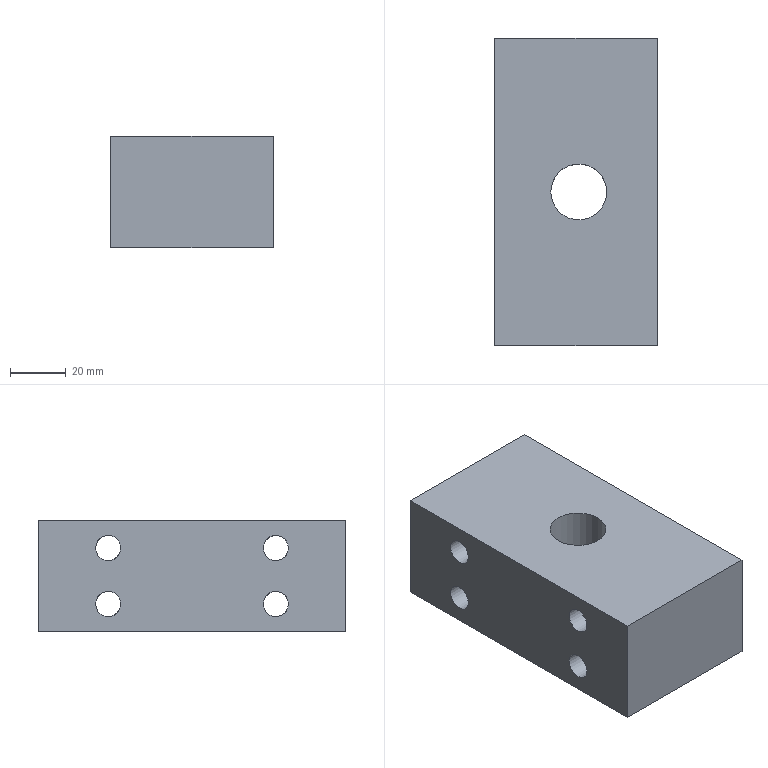Component | NX | CH3404_2-3 | 1 solid | 11 faces | box 58 x 110 x 40 mm | volume 227874 mm3 | plane 6 | cylinder 5 | commonest cylinder face diameters 9 x4 20 x1
STEP:
#1=CARTESIAN_POINT('',(0.,0.,0.));
#2=DIRECTION('',(0.,0.,1.));
#3=DIRECTION('',(1.,0.,0.));
#4=AXIS2_PLACEMENT_3D('',#1,#2,#3);
#5=CARTESIAN_POINT('',(0.,30.,5.5));
#6=VERTEX_POINT('',#5);
#7=CARTESIAN_POINT('',(0.,30.,10.));
#8=DIRECTION('',(1.,0.,0.));
#9=DIRECTION('',(0.,0.,-1.));
#10=AXIS2_PLACEMENT_3D('',#7,#8,#9);
#11=CIRCLE('',#10,4.5);
#12=CARTESIAN_POINT('',(-0.,55.,20.));
#13=DIRECTION('',(1.,0.,0.));
#14=DIRECTION('',(0.,0.,-1.));
#15=AXIS2_PLACEMENT_3D('',#12,#13,#14);
#16=PLANE('',#15);
#17=CARTESIAN_POINT('',(10.,-25.));
#18=DIRECTION('',(1.,0.));
#19=AXIS2_PLACEMENT_2D('',#17,#18);
#20=CIRCLE('',#19,4.5);
#21=(GEOMETRIC_REPRESENTATION_CONTEXT(2)PARAMETRIC_REPRESENTATION_CONTEXT()REPRESENTATION_CONTEXT('',''));
#22=DEFINITIONAL_REPRESENTATION('',(#20),#21);
#23=PCURVE('',#16,#22);
#24=CARTESIAN_POINT('',(0.,30.,10.));
#25=DIRECTION('',(1.,0.,0.));
#26=DIRECTION('',(0.,0.,-1.));
#27=AXIS2_PLACEMENT_3D('',#24,#25,#26);
#28=CYLINDRICAL_SURFACE('',#27,4.5);
#29=CARTESIAN_POINT('',(0.,0.));
#30=DIRECTION('',(1.,0.));
#31=VECTOR('',#30,1.);
#32=LINE('',#29,#31);
#33=(GEOMETRIC_REPRESENTATION_CONTEXT(2)PARAMETRIC_REPRESENTATION_CONTEXT()REPRESENTATION_CONTEXT('',''));
#34=DEFINITIONAL_REPRESENTATION('',(#32),#33);
#35=PCURVE('',#28,#34);
#36=SURFACE_CURVE('',#11,(#23,#35),.PCURVE_S1.);
#37=EDGE_CURVE('',#6,#6,#36,.T.);
#38=ORIENTED_EDGE('',*,*,#37,.T.);
#39=EDGE_LOOP('',(#38));
#40=FACE_BOUND('',#39,.T.);
#41=CARTESIAN_POINT('',(0.,30.,-14.5));
#42=VERTEX_POINT('',#41);
#43=CARTESIAN_POINT('',(0.,30.,-10.));
#44=DIRECTION('',(1.,0.,0.));
#45=DIRECTION('',(0.,0.,-1.));
#46=AXIS2_PLACEMENT_3D('',#43,#44,#45);
#47=CIRCLE('',#46,4.5);
#48=CARTESIAN_POINT('',(30.,-25.));
#49=DIRECTION('',(1.,0.));
#50=AXIS2_PLACEMENT_2D('',#48,#49);
#51=CIRCLE('',#50,4.5);
#52=(GEOMETRIC_REPRESENTATION_CONTEXT(2)PARAMETRIC_REPRESENTATION_CONTEXT()REPRESENTATION_CONTEXT('',''));
#53=DEFINITIONAL_REPRESENTATION('',(#51),#52);
#54=PCURVE('',#16,#53);
#55=CARTESIAN_POINT('',(0.,30.,-10.));
#56=DIRECTION('',(1.,0.,0.));
#57=DIRECTION('',(0.,0.,-1.));
#58=AXIS2_PLACEMENT_3D('',#55,#56,#57);
#59=CYLINDRICAL_SURFACE('',#58,4.5);
#60=CARTESIAN_POINT('',(0.,0.));
#61=DIRECTION('',(1.,0.));
#62=VECTOR('',#61,1.);
#63=LINE('',#60,#62);
#64=(GEOMETRIC_REPRESENTATION_CONTEXT(2)PARAMETRIC_REPRESENTATION_CONTEXT()REPRESENTATION_CONTEXT('',''));
#65=DEFINITIONAL_REPRESENTATION('',(#63),#64);
#66=PCURVE('',#59,#65);
#67=SURFACE_CURVE('',#47,(#54,#66),.PCURVE_S1.);
#68=EDGE_CURVE('',#42,#42,#67,.T.);
#69=ORIENTED_EDGE('',*,*,#68,.T.);
#70=EDGE_LOOP('',(#69));
#71=FACE_BOUND('',#70,.T.);
#72=CARTESIAN_POINT('',(0.,-30.,5.5));
#73=VERTEX_POINT('',#72);
#74=CARTESIAN_POINT('',(0.,-30.,10.));
#75=DIRECTION('',(1.,0.,0.));
#76=DIRECTION('',(0.,0.,-1.));
#77=AXIS2_PLACEMENT_3D('',#74,#75,#76);
#78=CIRCLE('',#77,4.5);
#79=CARTESIAN_POINT('',(10.,-85.));
#80=DIRECTION('',(1.,0.));
#81=AXIS2_PLACEMENT_2D('',#79,#80);
#82=CIRCLE('',#81,4.5);
#83=(GEOMETRIC_REPRESENTATION_CONTEXT(2)PARAMETRIC_REPRESENTATION_CONTEXT()REPRESENTATION_CONTEXT('',''));
#84=DEFINITIONAL_REPRESENTATION('',(#82),#83);
#85=PCURVE('',#16,#84);
#86=CARTESIAN_POINT('',(0.,-30.,10.));
#87=DIRECTION('',(1.,0.,0.));
#88=DIRECTION('',(0.,0.,-1.));
#89=AXIS2_PLACEMENT_3D('',#86,#87,#88);
#90=CYLINDRICAL_SURFACE('',#89,4.5);
#91=CARTESIAN_POINT('',(0.,0.));
#92=DIRECTION('',(1.,0.));
#93=VECTOR('',#92,1.);
#94=LINE('',#91,#93);
#95=(GEOMETRIC_REPRESENTATION_CONTEXT(2)PARAMETRIC_REPRESENTATION_CONTEXT()REPRESENTATION_CONTEXT('',''));
#96=DEFINITIONAL_REPRESENTATION('',(#94),#95);
#97=PCURVE('',#90,#96);
#98=SURFACE_CURVE('',#78,(#85,#97),.PCURVE_S1.);
#99=EDGE_CURVE('',#73,#73,#98,.T.);
#100=ORIENTED_EDGE('',*,*,#99,.T.);
#101=EDGE_LOOP('',(#100));
#102=FACE_BOUND('',#101,.T.);
#103=CARTESIAN_POINT('',(0.,-30.,-14.5));
#104=VERTEX_POINT('',#103);
#105=CARTESIAN_POINT('',(0.,-30.,-10.));
#106=DIRECTION('',(1.,0.,0.));
#107=DIRECTION('',(0.,0.,-1.));
#108=AXIS2_PLACEMENT_3D('',#105,#106,#107);
#109=CIRCLE('',#108,4.5);
#110=CARTESIAN_POINT('',(30.,-85.));
#111=DIRECTION('',(1.,0.));
#112=AXIS2_PLACEMENT_2D('',#110,#111);
#113=CIRCLE('',#112,4.5);
#114=(GEOMETRIC_REPRESENTATION_CONTEXT(2)PARAMETRIC_REPRESENTATION_CONTEXT()REPRESENTATION_CONTEXT('',''));
#115=DEFINITIONAL_REPRESENTATION('',(#113),#114);
#116=PCURVE('',#16,#115);
#117=CARTESIAN_POINT('',(0.,-30.,-10.));
#118=DIRECTION('',(1.,0.,0.));
#119=DIRECTION('',(0.,0.,-1.));
#120=AXIS2_PLACEMENT_3D('',#117,#118,#119);
#121=CYLINDRICAL_SURFACE('',#120,4.5);
#122=CARTESIAN_POINT('',(0.,0.));
#123=DIRECTION('',(1.,0.));
#124=VECTOR('',#123,1.);
#125=LINE('',#122,#124);
#126=(GEOMETRIC_REPRESENTATION_CONTEXT(2)PARAMETRIC_REPRESENTATION_CONTEXT()REPRESENTATION_CONTEXT('',''));
#127=DEFINITIONAL_REPRESENTATION('',(#125),#126);
#128=PCURVE('',#121,#127);
#129=SURFACE_CURVE('',#109,(#116,#128),.PCURVE_S1.);
#130=EDGE_CURVE('',#104,#104,#129,.T.);
#131=ORIENTED_EDGE('',*,*,#130,.T.);
#132=EDGE_LOOP('',(#131));
#133=FACE_BOUND('',#132,.T.);
#134=CARTESIAN_POINT('',(-0.,55.,-20.));
#135=VERTEX_POINT('',#134);
#136=CARTESIAN_POINT('',(-0.,-55.,-20.));
#137=VERTEX_POINT('',#136);
#138=CARTESIAN_POINT('',(-0.,55.,-20.));
#139=DIRECTION('',(0.,-1.,0.));
#140=VECTOR('',#139,1.);
#141=LINE('',#138,#140);
#142=CARTESIAN_POINT('',(40.,0.));
#143=DIRECTION('',(0.,-1.));
#144=VECTOR('',#143,1.);
#145=LINE('',#142,#144);
#146=(GEOMETRIC_REPRESENTATION_CONTEXT(2)PARAMETRIC_REPRESENTATION_CONTEXT()REPRESENTATION_CONTEXT('',''));
#147=DEFINITIONAL_REPRESENTATION('',(#145),#146);
#148=PCURVE('',#16,#147);
#149=CARTESIAN_POINT('',(30.,-0.,-20.));
#150=DIRECTION('',(0.,0.,1.));
#151=DIRECTION('',(1.,0.,0.));
#152=AXIS2_PLACEMENT_3D('',#149,#150,#151);
#153=PLANE('',#152);
#154=CARTESIAN_POINT('',(-30.,55.));
#155=DIRECTION('',(0.,-1.));
#156=VECTOR('',#155,1.);
#157=LINE('',#154,#156);
#158=(GEOMETRIC_REPRESENTATION_CONTEXT(2)PARAMETRIC_REPRESENTATION_CONTEXT()REPRESENTATION_CONTEXT('',''));
#159=DEFINITIONAL_REPRESENTATION('',(#157),#158);
#160=PCURVE('',#153,#159);
#161=SURFACE_CURVE('',#141,(#148,#160),.PCURVE_S1.);
#162=EDGE_CURVE('',#135,#137,#161,.T.);
#163=ORIENTED_EDGE('',*,*,#162,.T.);
#164=CARTESIAN_POINT('',(-0.,-55.,20.));
#165=VERTEX_POINT('',#164);
#166=CARTESIAN_POINT('',(-0.,-55.,20.));
#167=DIRECTION('',(0.,0.,-1.));
#168=VECTOR('',#167,1.);
#169=LINE('',#166,#168);
#170=CARTESIAN_POINT('',(0.,-110.));
#171=DIRECTION('',(1.,0.));
#172=VECTOR('',#171,1.);
#173=LINE('',#170,#172);
#174=(GEOMETRIC_REPRESENTATION_CONTEXT(2)PARAMETRIC_REPRESENTATION_CONTEXT()REPRESENTATION_CONTEXT('',''));
#175=DEFINITIONAL_REPRESENTATION('',(#173),#174);
#176=PCURVE('',#16,#175);
#177=CARTESIAN_POINT('',(-0.,-55.,20.));
#178=DIRECTION('',(0.,1.,0.));
#179=DIRECTION('',(-1.,0.,0.));
#180=AXIS2_PLACEMENT_3D('',#177,#178,#179);
#181=PLANE('',#180);
#182=CARTESIAN_POINT('',(0.,0.));
#183=DIRECTION('',(0.,-1.));
#184=VECTOR('',#183,1.);
#185=LINE('',#182,#184);
#186=(GEOMETRIC_REPRESENTATION_CONTEXT(2)PARAMETRIC_REPRESENTATION_CONTEXT()REPRESENTATION_CONTEXT('',''));
#187=DEFINITIONAL_REPRESENTATION('',(#185),#186);
#188=PCURVE('',#181,#187);
#189=SURFACE_CURVE('',#169,(#176,#188),.PCURVE_S1.);
#190=EDGE_CURVE('',#165,#137,#189,.T.);
#191=ORIENTED_EDGE('',*,*,#190,.F.);
#192=CARTESIAN_POINT('',(-0.,55.,20.));
#193=VERTEX_POINT('',#192);
#194=CARTESIAN_POINT('',(-0.,55.,20.));
#195=DIRECTION('',(0.,-1.,0.));
#196=VECTOR('',#195,1.);
#197=LINE('',#194,#196);
#198=CARTESIAN_POINT('',(0.,0.));
#199=DIRECTION('',(0.,-1.));
#200=VECTOR('',#199,1.);
#201=LINE('',#198,#200);
#202=(GEOMETRIC_REPRESENTATION_CONTEXT(2)PARAMETRIC_REPRESENTATION_CONTEXT()REPRESENTATION_CONTEXT('',''));
#203=DEFINITIONAL_REPRESENTATION('',(#201),#202);
#204=PCURVE('',#16,#203);
#205=CARTESIAN_POINT('',(30.,-0.,20.));
#206=DIRECTION('',(0.,0.,1.));
#207=DIRECTION('',(1.,0.,0.));
#208=AXIS2_PLACEMENT_3D('',#205,#206,#207);
#209=PLANE('',#208);
#210=CARTESIAN_POINT('',(-30.,55.));
#211=DIRECTION('',(0.,-1.));
#212=VECTOR('',#211,1.);
#213=LINE('',#210,#212);
#214=(GEOMETRIC_REPRESENTATION_CONTEXT(2)PARAMETRIC_REPRESENTATION_CONTEXT()REPRESENTATION_CONTEXT('',''));
#215=DEFINITIONAL_REPRESENTATION('',(#213),#214);
#216=PCURVE('',#209,#215);
#217=SURFACE_CURVE('',#197,(#204,#216),.PCURVE_S1.);
#218=EDGE_CURVE('',#193,#165,#217,.T.);
#219=ORIENTED_EDGE('',*,*,#218,.F.);
#220=CARTESIAN_POINT('',(-0.,55.,20.));
#221=DIRECTION('',(0.,0.,-1.));
#222=VECTOR('',#221,1.);
#223=LINE('',#220,#222);
#224=CARTESIAN_POINT('',(0.,0.));
#225=DIRECTION('',(1.,0.));
#226=VECTOR('',#225,1.);
#227=LINE('',#224,#226);
#228=(GEOMETRIC_REPRESENTATION_CONTEXT(2)PARAMETRIC_REPRESENTATION_CONTEXT()REPRESENTATION_CONTEXT('',''));
#229=DEFINITIONAL_REPRESENTATION('',(#227),#228);
#230=PCURVE('',#16,#229);
#231=CARTESIAN_POINT('',(58.,55.,20.));
#232=DIRECTION('',(0.,-1.,0.));
#233=DIRECTION('',(0.,0.,-1.));
#234=AXIS2_PLACEMENT_3D('',#231,#232,#233);
#235=PLANE('',#234);
#236=CARTESIAN_POINT('',(0.,-58.));
#237=DIRECTION('',(1.,0.));
#238=VECTOR('',#237,1.);
#239=LINE('',#236,#238);
#240=(GEOMETRIC_REPRESENTATION_CONTEXT(2)PARAMETRIC_REPRESENTATION_CONTEXT()REPRESENTATION_CONTEXT('',''));
#241=DEFINITIONAL_REPRESENTATION('',(#239),#240);
#242=PCURVE('',#235,#241);
#243=SURFACE_CURVE('',#223,(#230,#242),.PCURVE_S1.);
#244=EDGE_CURVE('',#193,#135,#243,.T.);
#245=ORIENTED_EDGE('',*,*,#244,.T.);
#246=EDGE_LOOP('',(#163,#191,#219,#245));
#247=FACE_BOUND('',#246,.T.);
#248=ADVANCED_FACE('',(#40,#71,#102,#133,#247),#16,.F.);
#249=CARTESIAN_POINT('',(58.,-55.,-20.));
#250=VERTEX_POINT('',#249);
#251=CARTESIAN_POINT('',(-0.,-55.,-20.));
#252=DIRECTION('',(1.,-0.,0.));
#253=VECTOR('',#252,1.);
#254=LINE('',#251,#253);
#255=CARTESIAN_POINT('',(0.,-40.));
#256=DIRECTION('',(-1.,0.));
#257=VECTOR('',#256,1.);
#258=LINE('',#255,#257);
#259=(GEOMETRIC_REPRESENTATION_CONTEXT(2)PARAMETRIC_REPRESENTATION_CONTEXT()REPRESENTATION_CONTEXT('',''));
#260=DEFINITIONAL_REPRESENTATION('',(#258),#259);
#261=PCURVE('',#181,#260);
#262=CARTESIAN_POINT('',(-30.,-55.));
#263=DIRECTION('',(1.,-0.));
#264=VECTOR('',#263,1.);
#265=LINE('',#262,#264);
#266=(GEOMETRIC_REPRESENTATION_CONTEXT(2)PARAMETRIC_REPRESENTATION_CONTEXT()REPRESENTATION_CONTEXT('',''));
#267=DEFINITIONAL_REPRESENTATION('',(#265),#266);
#268=PCURVE('',#153,#267);
#269=SURFACE_CURVE('',#254,(#261,#268),.PCURVE_S1.);
#270=EDGE_CURVE('',#137,#250,#269,.T.);
#271=ORIENTED_EDGE('',*,*,#270,.T.);
#272=CARTESIAN_POINT('',(58.,-55.,20.));
#273=VERTEX_POINT('',#272);
#274=CARTESIAN_POINT('',(58.,-55.,20.));
#275=DIRECTION('',(0.,0.,-1.));
#276=VECTOR('',#275,1.);
#277=LINE('',#274,#276);
#278=CARTESIAN_POINT('',(-58.,0.));
#279=DIRECTION('',(0.,-1.));
#280=VECTOR('',#279,1.);
#281=LINE('',#278,#280);
#282=(GEOMETRIC_REPRESENTATION_CONTEXT(2)PARAMETRIC_REPRESENTATION_CONTEXT()REPRESENTATION_CONTEXT('',''));
#283=DEFINITIONAL_REPRESENTATION('',(#281),#282);
#284=PCURVE('',#181,#283);
#285=CARTESIAN_POINT('',(58.,-55.,20.));
#286=DIRECTION('',(-1.,0.,0.));
#287=DIRECTION('',(-0.,-1.,0.));
#288=AXIS2_PLACEMENT_3D('',#285,#286,#287);
#289=PLANE('',#288);
#290=CARTESIAN_POINT('',(0.,0.));
#291=DIRECTION('',(0.,-1.));
#292=VECTOR('',#291,1.);
#293=LINE('',#290,#292);
#294=(GEOMETRIC_REPRESENTATION_CONTEXT(2)PARAMETRIC_REPRESENTATION_CONTEXT()REPRESENTATION_CONTEXT('',''));
#295=DEFINITIONAL_REPRESENTATION('',(#293),#294);
#296=PCURVE('',#289,#295);
#297=SURFACE_CURVE('',#277,(#284,#296),.PCURVE_S1.);
#298=EDGE_CURVE('',#273,#250,#297,.T.);
#299=ORIENTED_EDGE('',*,*,#298,.F.);
#300=CARTESIAN_POINT('',(-0.,-55.,20.));
#301=DIRECTION('',(1.,-0.,0.));
#302=VECTOR('',#301,1.);
#303=LINE('',#300,#302);
#304=CARTESIAN_POINT('',(0.,0.));
#305=DIRECTION('',(-1.,0.));
#306=VECTOR('',#305,1.);
#307=LINE('',#304,#306);
#308=(GEOMETRIC_REPRESENTATION_CONTEXT(2)PARAMETRIC_REPRESENTATION_CONTEXT()REPRESENTATION_CONTEXT('',''));
#309=DEFINITIONAL_REPRESENTATION('',(#307),#308);
#310=PCURVE('',#181,#309);
#311=CARTESIAN_POINT('',(-30.,-55.));
#312=DIRECTION('',(1.,-0.));
#313=VECTOR('',#312,1.);
#314=LINE('',#311,#313);
#315=(GEOMETRIC_REPRESENTATION_CONTEXT(2)PARAMETRIC_REPRESENTATION_CONTEXT()REPRESENTATION_CONTEXT('',''));
#316=DEFINITIONAL_REPRESENTATION('',(#314),#315);
#317=PCURVE('',#209,#316);
#318=SURFACE_CURVE('',#303,(#310,#317),.PCURVE_S1.);
#319=EDGE_CURVE('',#165,#273,#318,.T.);
#320=ORIENTED_EDGE('',*,*,#319,.F.);
#321=ORIENTED_EDGE('',*,*,#190,.T.);
#322=EDGE_LOOP('',(#271,#299,#320,#321));
#323=FACE_BOUND('',#322,.T.);
#324=ADVANCED_FACE('',(#323),#181,.F.);
#325=CARTESIAN_POINT('',(58.,25.5,10.));
#326=VERTEX_POINT('',#325);
#327=CARTESIAN_POINT('',(58.,30.,5.5));
#328=VERTEX_POINT('',#327);
#329=CARTESIAN_POINT('',(58.,30.,10.));
#330=DIRECTION('',(-1.,0.,0.));
#331=DIRECTION('',(-0.,-1.,0.));
#332=AXIS2_PLACEMENT_3D('',#329,#330,#331);
#333=CIRCLE('',#332,4.5);
#334=CARTESIAN_POINT('',(-85.,-10.));
#335=DIRECTION('',(1.,0.));
#336=AXIS2_PLACEMENT_2D('',#334,#335);
#337=CIRCLE('',#336,4.5);
#338=(GEOMETRIC_REPRESENTATION_CONTEXT(2)PARAMETRIC_REPRESENTATION_CONTEXT()REPRESENTATION_CONTEXT('',''));
#339=DEFINITIONAL_REPRESENTATION('',(#337),#338);
#340=PCURVE('',#289,#339);
#341=CARTESIAN_POINT('',(4.712,58.));
#342=DIRECTION('',(-1.,0.));
#343=VECTOR('',#342,1.);
#344=LINE('',#341,#343);
#345=(GEOMETRIC_REPRESENTATION_CONTEXT(2)PARAMETRIC_REPRESENTATION_CONTEXT()REPRESENTATION_CONTEXT('',''));
#346=DEFINITIONAL_REPRESENTATION('',(#344),#345);
#347=PCURVE('',#28,#346);
#348=SURFACE_CURVE('',#333,(#340,#347),.PCURVE_S1.);
#349=EDGE_CURVE('',#326,#328,#348,.T.);
#350=ORIENTED_EDGE('',*,*,#349,.T.);
#351=CARTESIAN_POINT('',(58.,30.,10.));
#352=DIRECTION('',(-1.,0.,0.));
#353=DIRECTION('',(-0.,-1.,0.));
#354=AXIS2_PLACEMENT_3D('',#351,#352,#353);
#355=CIRCLE('',#354,4.5);
#356=CARTESIAN_POINT('',(-85.,-10.));
#357=DIRECTION('',(1.,0.));
#358=AXIS2_PLACEMENT_2D('',#356,#357);
#359=CIRCLE('',#358,4.5);
#360=(GEOMETRIC_REPRESENTATION_CONTEXT(2)PARAMETRIC_REPRESENTATION_CONTEXT()REPRESENTATION_CONTEXT('',''));
#361=DEFINITIONAL_REPRESENTATION('',(#359),#360);
#362=PCURVE('',#289,#361);
#363=CARTESIAN_POINT('',(10.996,58.));
#364=DIRECTION('',(-1.,0.));
#365=VECTOR('',#364,1.);
#366=LINE('',#363,#365);
#367=(GEOMETRIC_REPRESENTATION_CONTEXT(2)PARAMETRIC_REPRESENTATION_CONTEXT()REPRESENTATION_CONTEXT('',''));
#368=DEFINITIONAL_REPRESENTATION('',(#366),#367);
#369=PCURVE('',#28,#368);
#370=SURFACE_CURVE('',#355,(#362,#369),.PCURVE_S1.);
#371=EDGE_CURVE('',#328,#326,#370,.T.);
#372=ORIENTED_EDGE('',*,*,#371,.T.);
#373=EDGE_LOOP('',(#350,#372));
#374=FACE_BOUND('',#373,.T.);
#375=CARTESIAN_POINT('',(58.,25.5,-10.));
#376=VERTEX_POINT('',#375);
#377=CARTESIAN_POINT('',(58.,30.,-14.5));
#378=VERTEX_POINT('',#377);
#379=CARTESIAN_POINT('',(58.,30.,-10.));
#380=DIRECTION('',(-1.,0.,0.));
#381=DIRECTION('',(-0.,-1.,0.));
#382=AXIS2_PLACEMENT_3D('',#379,#380,#381);
#383=CIRCLE('',#382,4.5);
#384=CARTESIAN_POINT('',(-85.,-30.));
#385=DIRECTION('',(1.,0.));
#386=AXIS2_PLACEMENT_2D('',#384,#385);
#387=CIRCLE('',#386,4.5);
#388=(GEOMETRIC_REPRESENTATION_CONTEXT(2)PARAMETRIC_REPRESENTATION_CONTEXT()REPRESENTATION_CONTEXT('',''));
#389=DEFINITIONAL_REPRESENTATION('',(#387),#388);
#390=PCURVE('',#289,#389);
#391=CARTESIAN_POINT('',(4.712,58.));
#392=DIRECTION('',(-1.,0.));
#393=VECTOR('',#392,1.);
#394=LINE('',#391,#393);
#395=(GEOMETRIC_REPRESENTATION_CONTEXT(2)PARAMETRIC_REPRESENTATION_CONTEXT()REPRESENTATION_CONTEXT('',''));
#396=DEFINITIONAL_REPRESENTATION('',(#394),#395);
#397=PCURVE('',#59,#396);
#398=SURFACE_CURVE('',#383,(#390,#397),.PCURVE_S1.);
#399=EDGE_CURVE('',#376,#378,#398,.T.);
#400=ORIENTED_EDGE('',*,*,#399,.T.);
#401=CARTESIAN_POINT('',(58.,30.,-10.));
#402=DIRECTION('',(-1.,0.,0.));
#403=DIRECTION('',(-0.,-1.,0.));
#404=AXIS2_PLACEMENT_3D('',#401,#402,#403);
#405=CIRCLE('',#404,4.5);
#406=CARTESIAN_POINT('',(-85.,-30.));
#407=DIRECTION('',(1.,0.));
#408=AXIS2_PLACEMENT_2D('',#406,#407);
#409=CIRCLE('',#408,4.5);
#410=(GEOMETRIC_REPRESENTATION_CONTEXT(2)PARAMETRIC_REPRESENTATION_CONTEXT()REPRESENTATION_CONTEXT('',''));
#411=DEFINITIONAL_REPRESENTATION('',(#409),#410);
#412=PCURVE('',#289,#411);
#413=CARTESIAN_POINT('',(10.996,58.));
#414=DIRECTION('',(-1.,0.));
#415=VECTOR('',#414,1.);
#416=LINE('',#413,#415);
#417=(GEOMETRIC_REPRESENTATION_CONTEXT(2)PARAMETRIC_REPRESENTATION_CONTEXT()REPRESENTATION_CONTEXT('',''));
#418=DEFINITIONAL_REPRESENTATION('',(#416),#417);
#419=PCURVE('',#59,#418);
#420=SURFACE_CURVE('',#405,(#412,#419),.PCURVE_S1.);
#421=EDGE_CURVE('',#378,#376,#420,.T.);
#422=ORIENTED_EDGE('',*,*,#421,.T.);
#423=EDGE_LOOP('',(#400,#422));
#424=FACE_BOUND('',#423,.T.);
#425=CARTESIAN_POINT('',(58.,-34.5,10.));
#426=VERTEX_POINT('',#425);
#427=CARTESIAN_POINT('',(58.,-30.,5.5));
#428=VERTEX_POINT('',#427);
#429=CARTESIAN_POINT('',(58.,-30.,10.));
#430=DIRECTION('',(-1.,0.,0.));
#431=DIRECTION('',(-0.,-1.,0.));
#432=AXIS2_PLACEMENT_3D('',#429,#430,#431);
#433=CIRCLE('',#432,4.5);
#434=CARTESIAN_POINT('',(-25.,-10.));
#435=DIRECTION('',(1.,0.));
#436=AXIS2_PLACEMENT_2D('',#434,#435);
#437=CIRCLE('',#436,4.5);
#438=(GEOMETRIC_REPRESENTATION_CONTEXT(2)PARAMETRIC_REPRESENTATION_CONTEXT()REPRESENTATION_CONTEXT('',''));
#439=DEFINITIONAL_REPRESENTATION('',(#437),#438);
#440=PCURVE('',#289,#439);
#441=CARTESIAN_POINT('',(4.712,58.));
#442=DIRECTION('',(-1.,0.));
#443=VECTOR('',#442,1.);
#444=LINE('',#441,#443);
#445=(GEOMETRIC_REPRESENTATION_CONTEXT(2)PARAMETRIC_REPRESENTATION_CONTEXT()REPRESENTATION_CONTEXT('',''));
#446=DEFINITIONAL_REPRESENTATION('',(#444),#445);
#447=PCURVE('',#90,#446);
#448=SURFACE_CURVE('',#433,(#440,#447),.PCURVE_S1.);
#449=EDGE_CURVE('',#426,#428,#448,.T.);
#450=ORIENTED_EDGE('',*,*,#449,.T.);
#451=CARTESIAN_POINT('',(58.,-30.,10.));
#452=DIRECTION('',(-1.,0.,0.));
#453=DIRECTION('',(-0.,-1.,0.));
#454=AXIS2_PLACEMENT_3D('',#451,#452,#453);
#455=CIRCLE('',#454,4.5);
#456=CARTESIAN_POINT('',(-25.,-10.));
#457=DIRECTION('',(1.,0.));
#458=AXIS2_PLACEMENT_2D('',#456,#457);
#459=CIRCLE('',#458,4.5);
#460=(GEOMETRIC_REPRESENTATION_CONTEXT(2)PARAMETRIC_REPRESENTATION_CONTEXT()REPRESENTATION_CONTEXT('',''));
#461=DEFINITIONAL_REPRESENTATION('',(#459),#460);
#462=PCURVE('',#289,#461);
#463=CARTESIAN_POINT('',(10.996,58.));
#464=DIRECTION('',(-1.,0.));
#465=VECTOR('',#464,1.);
#466=LINE('',#463,#465);
#467=(GEOMETRIC_REPRESENTATION_CONTEXT(2)PARAMETRIC_REPRESENTATION_CONTEXT()REPRESENTATION_CONTEXT('',''));
#468=DEFINITIONAL_REPRESENTATION('',(#466),#467);
#469=PCURVE('',#90,#468);
#470=SURFACE_CURVE('',#455,(#462,#469),.PCURVE_S1.);
#471=EDGE_CURVE('',#428,#426,#470,.T.);
#472=ORIENTED_EDGE('',*,*,#471,.T.);
#473=EDGE_LOOP('',(#450,#472));
#474=FACE_BOUND('',#473,.T.);
#475=CARTESIAN_POINT('',(58.,-34.5,-10.));
#476=VERTEX_POINT('',#475);
#477=CARTESIAN_POINT('',(58.,-30.,-14.5));
#478=VERTEX_POINT('',#477);
#479=CARTESIAN_POINT('',(58.,-30.,-10.));
#480=DIRECTION('',(-1.,0.,0.));
#481=DIRECTION('',(-0.,-1.,0.));
#482=AXIS2_PLACEMENT_3D('',#479,#480,#481);
#483=CIRCLE('',#482,4.5);
#484=CARTESIAN_POINT('',(-25.,-30.));
#485=DIRECTION('',(1.,0.));
#486=AXIS2_PLACEMENT_2D('',#484,#485);
#487=CIRCLE('',#486,4.5);
#488=(GEOMETRIC_REPRESENTATION_CONTEXT(2)PARAMETRIC_REPRESENTATION_CONTEXT()REPRESENTATION_CONTEXT('',''));
#489=DEFINITIONAL_REPRESENTATION('',(#487),#488);
#490=PCURVE('',#289,#489);
#491=CARTESIAN_POINT('',(4.712,58.));
#492=DIRECTION('',(-1.,0.));
#493=VECTOR('',#492,1.);
#494=LINE('',#491,#493);
#495=(GEOMETRIC_REPRESENTATION_CONTEXT(2)PARAMETRIC_REPRESENTATION_CONTEXT()REPRESENTATION_CONTEXT('',''));
#496=DEFINITIONAL_REPRESENTATION('',(#494),#495);
#497=PCURVE('',#121,#496);
#498=SURFACE_CURVE('',#483,(#490,#497),.PCURVE_S1.);
#499=EDGE_CURVE('',#476,#478,#498,.T.);
#500=ORIENTED_EDGE('',*,*,#499,.T.);
#501=CARTESIAN_POINT('',(58.,-30.,-10.));
#502=DIRECTION('',(-1.,0.,0.));
#503=DIRECTION('',(-0.,-1.,0.));
#504=AXIS2_PLACEMENT_3D('',#501,#502,#503);
#505=CIRCLE('',#504,4.5);
#506=CARTESIAN_POINT('',(-25.,-30.));
#507=DIRECTION('',(1.,0.));
#508=AXIS2_PLACEMENT_2D('',#506,#507);
#509=CIRCLE('',#508,4.5);
#510=(GEOMETRIC_REPRESENTATION_CONTEXT(2)PARAMETRIC_REPRESENTATION_CONTEXT()REPRESENTATION_CONTEXT('',''));
#511=DEFINITIONAL_REPRESENTATION('',(#509),#510);
#512=PCURVE('',#289,#511);
#513=CARTESIAN_POINT('',(10.996,58.));
#514=DIRECTION('',(-1.,0.));
#515=VECTOR('',#514,1.);
#516=LINE('',#513,#515);
#517=(GEOMETRIC_REPRESENTATION_CONTEXT(2)PARAMETRIC_REPRESENTATION_CONTEXT()REPRESENTATION_CONTEXT('',''));
#518=DEFINITIONAL_REPRESENTATION('',(#516),#517);
#519=PCURVE('',#121,#518);
#520=SURFACE_CURVE('',#505,(#512,#519),.PCURVE_S1.);
#521=EDGE_CURVE('',#478,#476,#520,.T.);
#522=ORIENTED_EDGE('',*,*,#521,.T.);
#523=EDGE_LOOP('',(#500,#522));
#524=FACE_BOUND('',#523,.T.);
#525=CARTESIAN_POINT('',(58.,55.,-20.));
#526=VERTEX_POINT('',#525);
#527=CARTESIAN_POINT('',(58.,-55.,-20.));
#528=DIRECTION('',(0.,1.,0.));
#529=VECTOR('',#528,1.);
#530=LINE('',#527,#529);
#531=CARTESIAN_POINT('',(0.,-40.));
#532=DIRECTION('',(-1.,0.));
#533=VECTOR('',#532,1.);
#534=LINE('',#531,#533);
#535=(GEOMETRIC_REPRESENTATION_CONTEXT(2)PARAMETRIC_REPRESENTATION_CONTEXT()REPRESENTATION_CONTEXT('',''));
#536=DEFINITIONAL_REPRESENTATION('',(#534),#535);
#537=PCURVE('',#289,#536);
#538=CARTESIAN_POINT('',(28.,-55.));
#539=DIRECTION('',(0.,1.));
#540=VECTOR('',#539,1.);
#541=LINE('',#538,#540);
#542=(GEOMETRIC_REPRESENTATION_CONTEXT(2)PARAMETRIC_REPRESENTATION_CONTEXT()REPRESENTATION_CONTEXT('',''));
#543=DEFINITIONAL_REPRESENTATION('',(#541),#542);
#544=PCURVE('',#153,#543);
#545=SURFACE_CURVE('',#530,(#537,#544),.PCURVE_S1.);
#546=EDGE_CURVE('',#250,#526,#545,.T.);
#547=ORIENTED_EDGE('',*,*,#546,.T.);
#548=CARTESIAN_POINT('',(58.,55.,20.));
#549=VERTEX_POINT('',#548);
#550=CARTESIAN_POINT('',(58.,55.,20.));
#551=DIRECTION('',(0.,0.,-1.));
#552=VECTOR('',#551,1.);
#553=LINE('',#550,#552);
#554=CARTESIAN_POINT('',(-110.,0.));
#555=DIRECTION('',(0.,-1.));
#556=VECTOR('',#555,1.);
#557=LINE('',#554,#556);
#558=(GEOMETRIC_REPRESENTATION_CONTEXT(2)PARAMETRIC_REPRESENTATION_CONTEXT()REPRESENTATION_CONTEXT('',''));
#559=DEFINITIONAL_REPRESENTATION('',(#557),#558);
#560=PCURVE('',#289,#559);
#561=CARTESIAN_POINT('',(0.,0.));
#562=DIRECTION('',(1.,0.));
#563=VECTOR('',#562,1.);
#564=LINE('',#561,#563);
#565=(GEOMETRIC_REPRESENTATION_CONTEXT(2)PARAMETRIC_REPRESENTATION_CONTEXT()REPRESENTATION_CONTEXT('',''));
#566=DEFINITIONAL_REPRESENTATION('',(#564),#565);
#567=PCURVE('',#235,#566);
#568=SURFACE_CURVE('',#553,(#560,#567),.PCURVE_S1.);
#569=EDGE_CURVE('',#549,#526,#568,.T.);
#570=ORIENTED_EDGE('',*,*,#569,.F.);
#571=CARTESIAN_POINT('',(58.,-55.,20.));
#572=DIRECTION('',(0.,1.,0.));
#573=VECTOR('',#572,1.);
#574=LINE('',#571,#573);
#575=CARTESIAN_POINT('',(0.,0.));
#576=DIRECTION('',(-1.,0.));
#577=VECTOR('',#576,1.);
#578=LINE('',#575,#577);
#579=(GEOMETRIC_REPRESENTATION_CONTEXT(2)PARAMETRIC_REPRESENTATION_CONTEXT()REPRESENTATION_CONTEXT('',''));
#580=DEFINITIONAL_REPRESENTATION('',(#578),#579);
#581=PCURVE('',#289,#580);
#582=CARTESIAN_POINT('',(28.,-55.));
#583=DIRECTION('',(0.,1.));
#584=VECTOR('',#583,1.);
#585=LINE('',#582,#584);
#586=(GEOMETRIC_REPRESENTATION_CONTEXT(2)PARAMETRIC_REPRESENTATION_CONTEXT()REPRESENTATION_CONTEXT('',''));
#587=DEFINITIONAL_REPRESENTATION('',(#585),#586);
#588=PCURVE('',#209,#587);
#589=SURFACE_CURVE('',#574,(#581,#588),.PCURVE_S1.);
#590=EDGE_CURVE('',#273,#549,#589,.T.);
#591=ORIENTED_EDGE('',*,*,#590,.F.);
#592=ORIENTED_EDGE('',*,*,#298,.T.);
#593=EDGE_LOOP('',(#547,#570,#591,#592));
#594=FACE_BOUND('',#593,.T.);
#595=ADVANCED_FACE('',(#374,#424,#474,#524,#594),#289,.F.);
#596=CARTESIAN_POINT('',(58.,55.,-20.));
#597=DIRECTION('',(-1.,0.,0.));
#598=VECTOR('',#597,1.);
#599=LINE('',#596,#598);
#600=CARTESIAN_POINT('',(40.,0.));
#601=DIRECTION('',(0.,-1.));
#602=VECTOR('',#601,1.);
#603=LINE('',#600,#602);
#604=(GEOMETRIC_REPRESENTATION_CONTEXT(2)PARAMETRIC_REPRESENTATION_CONTEXT()REPRESENTATION_CONTEXT('',''));
#605=DEFINITIONAL_REPRESENTATION('',(#603),#604);
#606=PCURVE('',#235,#605);
#607=CARTESIAN_POINT('',(28.,55.));
#608=DIRECTION('',(-1.,0.));
#609=VECTOR('',#608,1.);
#610=LINE('',#607,#609);
#611=(GEOMETRIC_REPRESENTATION_CONTEXT(2)PARAMETRIC_REPRESENTATION_CONTEXT()REPRESENTATION_CONTEXT('',''));
#612=DEFINITIONAL_REPRESENTATION('',(#610),#611);
#613=PCURVE('',#153,#612);
#614=SURFACE_CURVE('',#599,(#606,#613),.PCURVE_S1.);
#615=EDGE_CURVE('',#526,#135,#614,.T.);
#616=ORIENTED_EDGE('',*,*,#615,.T.);
#617=ORIENTED_EDGE('',*,*,#244,.F.);
#618=CARTESIAN_POINT('',(58.,55.,20.));
#619=DIRECTION('',(-1.,0.,0.));
#620=VECTOR('',#619,1.);
#621=LINE('',#618,#620);
#622=CARTESIAN_POINT('',(0.,0.));
#623=DIRECTION('',(0.,-1.));
#624=VECTOR('',#623,1.);
#625=LINE('',#622,#624);
#626=(GEOMETRIC_REPRESENTATION_CONTEXT(2)PARAMETRIC_REPRESENTATION_CONTEXT()REPRESENTATION_CONTEXT('',''));
#627=DEFINITIONAL_REPRESENTATION('',(#625),#626);
#628=PCURVE('',#235,#627);
#629=CARTESIAN_POINT('',(28.,55.));
#630=DIRECTION('',(-1.,0.));
#631=VECTOR('',#630,1.);
#632=LINE('',#629,#631);
#633=(GEOMETRIC_REPRESENTATION_CONTEXT(2)PARAMETRIC_REPRESENTATION_CONTEXT()REPRESENTATION_CONTEXT('',''));
#634=DEFINITIONAL_REPRESENTATION('',(#632),#633);
#635=PCURVE('',#209,#634);
#636=SURFACE_CURVE('',#621,(#628,#635),.PCURVE_S1.);
#637=EDGE_CURVE('',#549,#193,#636,.T.);
#638=ORIENTED_EDGE('',*,*,#637,.F.);
#639=ORIENTED_EDGE('',*,*,#569,.T.);
#640=EDGE_LOOP('',(#616,#617,#638,#639));
#641=FACE_BOUND('',#640,.T.);
#642=ADVANCED_FACE('',(#641),#235,.F.);
#643=CARTESIAN_POINT('',(40.,-0.,20.));
#644=VERTEX_POINT('',#643);
#645=CARTESIAN_POINT('',(30.,-0.,20.));
#646=DIRECTION('',(0.,0.,1.));
#647=DIRECTION('',(1.,0.,0.));
#648=AXIS2_PLACEMENT_3D('',#645,#646,#647);
#649=CIRCLE('',#648,10.);
#650=CARTESIAN_POINT('',(30.,-0.,20.));
#651=DIRECTION('',(0.,0.,-1.));
#652=DIRECTION('',(-1.,0.,0.));
#653=AXIS2_PLACEMENT_3D('',#650,#651,#652);
#654=CYLINDRICAL_SURFACE('',#653,10.);
#655=CARTESIAN_POINT('',(9.425,0.));
#656=DIRECTION('',(-1.,0.));
#657=VECTOR('',#656,1.);
#658=LINE('',#655,#657);
#659=(GEOMETRIC_REPRESENTATION_CONTEXT(2)PARAMETRIC_REPRESENTATION_CONTEXT()REPRESENTATION_CONTEXT('',''));
#660=DEFINITIONAL_REPRESENTATION('',(#658),#659);
#661=PCURVE('',#654,#660);
#662=CARTESIAN_POINT('',(0.,0.));
#663=DIRECTION('',(1.,0.));
#664=AXIS2_PLACEMENT_2D('',#662,#663);
#665=CIRCLE('',#664,10.);
#666=(GEOMETRIC_REPRESENTATION_CONTEXT(2)PARAMETRIC_REPRESENTATION_CONTEXT()REPRESENTATION_CONTEXT('',''));
#667=DEFINITIONAL_REPRESENTATION('',(#665),#666);
#668=PCURVE('',#209,#667);
#669=SURFACE_CURVE('',#649,(#661,#668),.PCURVE_S1.);
#670=EDGE_CURVE('',#644,#644,#669,.T.);
#671=ORIENTED_EDGE('',*,*,#670,.F.);
#672=CARTESIAN_POINT('',(40.,-0.,-20.));
#673=VERTEX_POINT('',#672);
#674=CARTESIAN_POINT('',(40.,-0.,20.));
#675=CARTESIAN_POINT('',(40.,-0.,-20.));
#676=B_SPLINE_CURVE_WITH_KNOTS('',1,(#674,#675),.UNSPECIFIED.,.F.,.F.,(2,2),(0.,40.),.PIECEWISE_BEZIER_KNOTS.);
#677=CARTESIAN_POINT('',(9.425,0.));
#678=DIRECTION('',(0.,1.));
#679=VECTOR('',#678,1.);
#680=LINE('',#677,#679);
#681=(GEOMETRIC_REPRESENTATION_CONTEXT(2)PARAMETRIC_REPRESENTATION_CONTEXT()REPRESENTATION_CONTEXT('',''));
#682=DEFINITIONAL_REPRESENTATION('',(#680),#681);
#683=PCURVE('',#654,#682);
#684=CARTESIAN_POINT('',(3.142,0.));
#685=DIRECTION('',(0.,1.));
#686=VECTOR('',#685,1.);
#687=LINE('',#684,#686);
#688=(GEOMETRIC_REPRESENTATION_CONTEXT(2)PARAMETRIC_REPRESENTATION_CONTEXT()REPRESENTATION_CONTEXT('',''));
#689=DEFINITIONAL_REPRESENTATION('',(#687),#688);
#690=PCURVE('',#654,#689);
#691=SEAM_CURVE('',#676,(#683,#690),.PCURVE_S1.);
#692=EDGE_CURVE('',#644,#673,#691,.T.);
#693=ORIENTED_EDGE('',*,*,#692,.T.);
#694=CARTESIAN_POINT('',(30.,-0.,-20.));
#695=DIRECTION('',(0.,0.,1.));
#696=DIRECTION('',(1.,0.,0.));
#697=AXIS2_PLACEMENT_3D('',#694,#695,#696);
#698=CIRCLE('',#697,10.);
#699=CARTESIAN_POINT('',(9.425,40.));
#700=DIRECTION('',(-1.,0.));
#701=VECTOR('',#700,1.);
#702=LINE('',#699,#701);
#703=(GEOMETRIC_REPRESENTATION_CONTEXT(2)PARAMETRIC_REPRESENTATION_CONTEXT()REPRESENTATION_CONTEXT('',''));
#704=DEFINITIONAL_REPRESENTATION('',(#702),#703);
#705=PCURVE('',#654,#704);
#706=CARTESIAN_POINT('',(0.,0.));
#707=DIRECTION('',(1.,0.));
#708=AXIS2_PLACEMENT_2D('',#706,#707);
#709=CIRCLE('',#708,10.);
#710=(GEOMETRIC_REPRESENTATION_CONTEXT(2)PARAMETRIC_REPRESENTATION_CONTEXT()REPRESENTATION_CONTEXT('',''));
#711=DEFINITIONAL_REPRESENTATION('',(#709),#710);
#712=PCURVE('',#153,#711);
#713=SURFACE_CURVE('',#698,(#705,#712),.PCURVE_S1.);
#714=EDGE_CURVE('',#673,#673,#713,.T.);
#715=ORIENTED_EDGE('',*,*,#714,.T.);
#716=ORIENTED_EDGE('',*,*,#692,.F.);
#717=EDGE_LOOP('',(#671,#693,#715,#716));
#718=FACE_BOUND('',#717,.F.);
#719=ADVANCED_FACE('',(#718),#654,.F.);
#720=ORIENTED_EDGE('',*,*,#218,.T.);
#721=ORIENTED_EDGE('',*,*,#319,.T.);
#722=ORIENTED_EDGE('',*,*,#590,.T.);
#723=ORIENTED_EDGE('',*,*,#637,.T.);
#724=EDGE_LOOP('',(#720,#721,#722,#723));
#725=FACE_BOUND('',#724,.T.);
#726=ORIENTED_EDGE('',*,*,#670,.F.);
#727=EDGE_LOOP('',(#726));
#728=FACE_BOUND('',#727,.T.);
#729=ADVANCED_FACE('',(#725,#728),#209,.T.);
#730=ORIENTED_EDGE('',*,*,#162,.F.);
#731=ORIENTED_EDGE('',*,*,#615,.F.);
#732=ORIENTED_EDGE('',*,*,#546,.F.);
#733=ORIENTED_EDGE('',*,*,#270,.F.);
#734=EDGE_LOOP('',(#730,#731,#732,#733));
#735=FACE_BOUND('',#734,.T.);
#736=ORIENTED_EDGE('',*,*,#714,.T.);
#737=EDGE_LOOP('',(#736));
#738=FACE_BOUND('',#737,.T.);
#739=ADVANCED_FACE('',(#735,#738),#153,.F.);
#740=ORIENTED_EDGE('',*,*,#130,.T.);
#741=CARTESIAN_POINT('',(0.,-30.,-14.5));
#742=CARTESIAN_POINT('',(58.,-30.,-14.5));
#743=B_SPLINE_CURVE_WITH_KNOTS('',1,(#741,#742),.UNSPECIFIED.,.F.,.F.,(2,2),(0.,58.),.PIECEWISE_BEZIER_KNOTS.);
#744=CARTESIAN_POINT('',(6.283,0.));
#745=DIRECTION('',(0.,1.));
#746=VECTOR('',#745,1.);
#747=LINE('',#744,#746);
#748=(GEOMETRIC_REPRESENTATION_CONTEXT(2)PARAMETRIC_REPRESENTATION_CONTEXT()REPRESENTATION_CONTEXT('',''));
#749=DEFINITIONAL_REPRESENTATION('',(#747),#748);
#750=PCURVE('',#121,#749);
#751=CARTESIAN_POINT('',(0.,0.));
#752=DIRECTION('',(0.,1.));
#753=VECTOR('',#752,1.);
#754=LINE('',#751,#753);
#755=(GEOMETRIC_REPRESENTATION_CONTEXT(2)PARAMETRIC_REPRESENTATION_CONTEXT()REPRESENTATION_CONTEXT('',''));
#756=DEFINITIONAL_REPRESENTATION('',(#754),#755);
#757=PCURVE('',#121,#756);
#758=SEAM_CURVE('',#743,(#750,#757),.PCURVE_S1.);
#759=EDGE_CURVE('',#104,#478,#758,.T.);
#760=ORIENTED_EDGE('',*,*,#759,.T.);
#761=ORIENTED_EDGE('',*,*,#521,.T.);
#762=ORIENTED_EDGE('',*,*,#499,.T.);
#763=ORIENTED_EDGE('',*,*,#759,.F.);
#764=EDGE_LOOP('',(#740,#760,#761,#762,#763));
#765=FACE_BOUND('',#764,.F.);
#766=ADVANCED_FACE('',(#765),#121,.F.);
#767=ORIENTED_EDGE('',*,*,#99,.T.);
#768=CARTESIAN_POINT('',(0.,-30.,5.5));
#769=CARTESIAN_POINT('',(58.,-30.,5.5));
#770=B_SPLINE_CURVE_WITH_KNOTS('',1,(#768,#769),.UNSPECIFIED.,.F.,.F.,(2,2),(0.,58.),.PIECEWISE_BEZIER_KNOTS.);
#771=CARTESIAN_POINT('',(6.283,0.));
#772=DIRECTION('',(0.,1.));
#773=VECTOR('',#772,1.);
#774=LINE('',#771,#773);
#775=(GEOMETRIC_REPRESENTATION_CONTEXT(2)PARAMETRIC_REPRESENTATION_CONTEXT()REPRESENTATION_CONTEXT('',''));
#776=DEFINITIONAL_REPRESENTATION('',(#774),#775);
#777=PCURVE('',#90,#776);
#778=CARTESIAN_POINT('',(0.,0.));
#779=DIRECTION('',(0.,1.));
#780=VECTOR('',#779,1.);
#781=LINE('',#778,#780);
#782=(GEOMETRIC_REPRESENTATION_CONTEXT(2)PARAMETRIC_REPRESENTATION_CONTEXT()REPRESENTATION_CONTEXT('',''));
#783=DEFINITIONAL_REPRESENTATION('',(#781),#782);
#784=PCURVE('',#90,#783);
#785=SEAM_CURVE('',#770,(#777,#784),.PCURVE_S1.);
#786=EDGE_CURVE('',#73,#428,#785,.T.);
#787=ORIENTED_EDGE('',*,*,#786,.T.);
#788=ORIENTED_EDGE('',*,*,#471,.T.);
#789=ORIENTED_EDGE('',*,*,#449,.T.);
#790=ORIENTED_EDGE('',*,*,#786,.F.);
#791=EDGE_LOOP('',(#767,#787,#788,#789,#790));
#792=FACE_BOUND('',#791,.F.);
#793=ADVANCED_FACE('',(#792),#90,.F.);
#794=ORIENTED_EDGE('',*,*,#68,.T.);
#795=CARTESIAN_POINT('',(0.,30.,-14.5));
#796=CARTESIAN_POINT('',(58.,30.,-14.5));
#797=B_SPLINE_CURVE_WITH_KNOTS('',1,(#795,#796),.UNSPECIFIED.,.F.,.F.,(2,2),(0.,58.),.PIECEWISE_BEZIER_KNOTS.);
#798=CARTESIAN_POINT('',(6.283,0.));
#799=DIRECTION('',(0.,1.));
#800=VECTOR('',#799,1.);
#801=LINE('',#798,#800);
#802=(GEOMETRIC_REPRESENTATION_CONTEXT(2)PARAMETRIC_REPRESENTATION_CONTEXT()REPRESENTATION_CONTEXT('',''));
#803=DEFINITIONAL_REPRESENTATION('',(#801),#802);
#804=PCURVE('',#59,#803);
#805=CARTESIAN_POINT('',(0.,0.));
#806=DIRECTION('',(0.,1.));
#807=VECTOR('',#806,1.);
#808=LINE('',#805,#807);
#809=(GEOMETRIC_REPRESENTATION_CONTEXT(2)PARAMETRIC_REPRESENTATION_CONTEXT()REPRESENTATION_CONTEXT('',''));
#810=DEFINITIONAL_REPRESENTATION('',(#808),#809);
#811=PCURVE('',#59,#810);
#812=SEAM_CURVE('',#797,(#804,#811),.PCURVE_S1.);
#813=EDGE_CURVE('',#42,#378,#812,.T.);
#814=ORIENTED_EDGE('',*,*,#813,.T.);
#815=ORIENTED_EDGE('',*,*,#421,.T.);
#816=ORIENTED_EDGE('',*,*,#399,.T.);
#817=ORIENTED_EDGE('',*,*,#813,.F.);
#818=EDGE_LOOP('',(#794,#814,#815,#816,#817));
#819=FACE_BOUND('',#818,.F.);
#820=ADVANCED_FACE('',(#819),#59,.F.);
#821=ORIENTED_EDGE('',*,*,#37,.T.);
#822=CARTESIAN_POINT('',(0.,30.,5.5));
#823=CARTESIAN_POINT('',(58.,30.,5.5));
#824=B_SPLINE_CURVE_WITH_KNOTS('',1,(#822,#823),.UNSPECIFIED.,.F.,.F.,(2,2),(0.,58.),.PIECEWISE_BEZIER_KNOTS.);
#825=CARTESIAN_POINT('',(6.283,0.));
#826=DIRECTION('',(0.,1.));
#827=VECTOR('',#826,1.);
#828=LINE('',#825,#827);
#829=(GEOMETRIC_REPRESENTATION_CONTEXT(2)PARAMETRIC_REPRESENTATION_CONTEXT()REPRESENTATION_CONTEXT('',''));
#830=DEFINITIONAL_REPRESENTATION('',(#828),#829);
#831=PCURVE('',#28,#830);
#832=CARTESIAN_POINT('',(0.,0.));
#833=DIRECTION('',(0.,1.));
#834=VECTOR('',#833,1.);
#835=LINE('',#832,#834);
#836=(GEOMETRIC_REPRESENTATION_CONTEXT(2)PARAMETRIC_REPRESENTATION_CONTEXT()REPRESENTATION_CONTEXT('',''));
#837=DEFINITIONAL_REPRESENTATION('',(#835),#836);
#838=PCURVE('',#28,#837);
#839=SEAM_CURVE('',#824,(#831,#838),.PCURVE_S1.);
#840=EDGE_CURVE('',#6,#328,#839,.T.);
#841=ORIENTED_EDGE('',*,*,#840,.T.);
#842=ORIENTED_EDGE('',*,*,#371,.T.);
#843=ORIENTED_EDGE('',*,*,#349,.T.);
#844=ORIENTED_EDGE('',*,*,#840,.F.);
#845=EDGE_LOOP('',(#821,#841,#842,#843,#844));
#846=FACE_BOUND('',#845,.F.);
#847=ADVANCED_FACE('',(#846),#28,.F.);
#848=CLOSED_SHELL('',(#248,#324,#595,#642,#719,#729,#739,#766,#793,#820,#847));
#849=MANIFOLD_SOLID_BREP('',#848);
#850=(LENGTH_UNIT()NAMED_UNIT(*)SI_UNIT(.MILLI.,.METRE.));
#851=UNCERTAINTY_MEASURE_WITH_UNIT(LENGTH_MEASURE(0.000005),#850,'','');
#852=(NAMED_UNIT(*)PLANE_ANGLE_UNIT()SI_UNIT($,.RADIAN.));
#853=(NAMED_UNIT(*)SI_UNIT($,.STERADIAN.)SOLID_ANGLE_UNIT());
#854=(GEOMETRIC_REPRESENTATION_CONTEXT(3)GLOBAL_UNCERTAINTY_ASSIGNED_CONTEXT((#851))GLOBAL_UNIT_ASSIGNED_CONTEXT((#850,#852,#853))REPRESENTATION_CONTEXT('',''));
#855=ADVANCED_BREP_SHAPE_REPRESENTATION('',(#4,#849),#854);